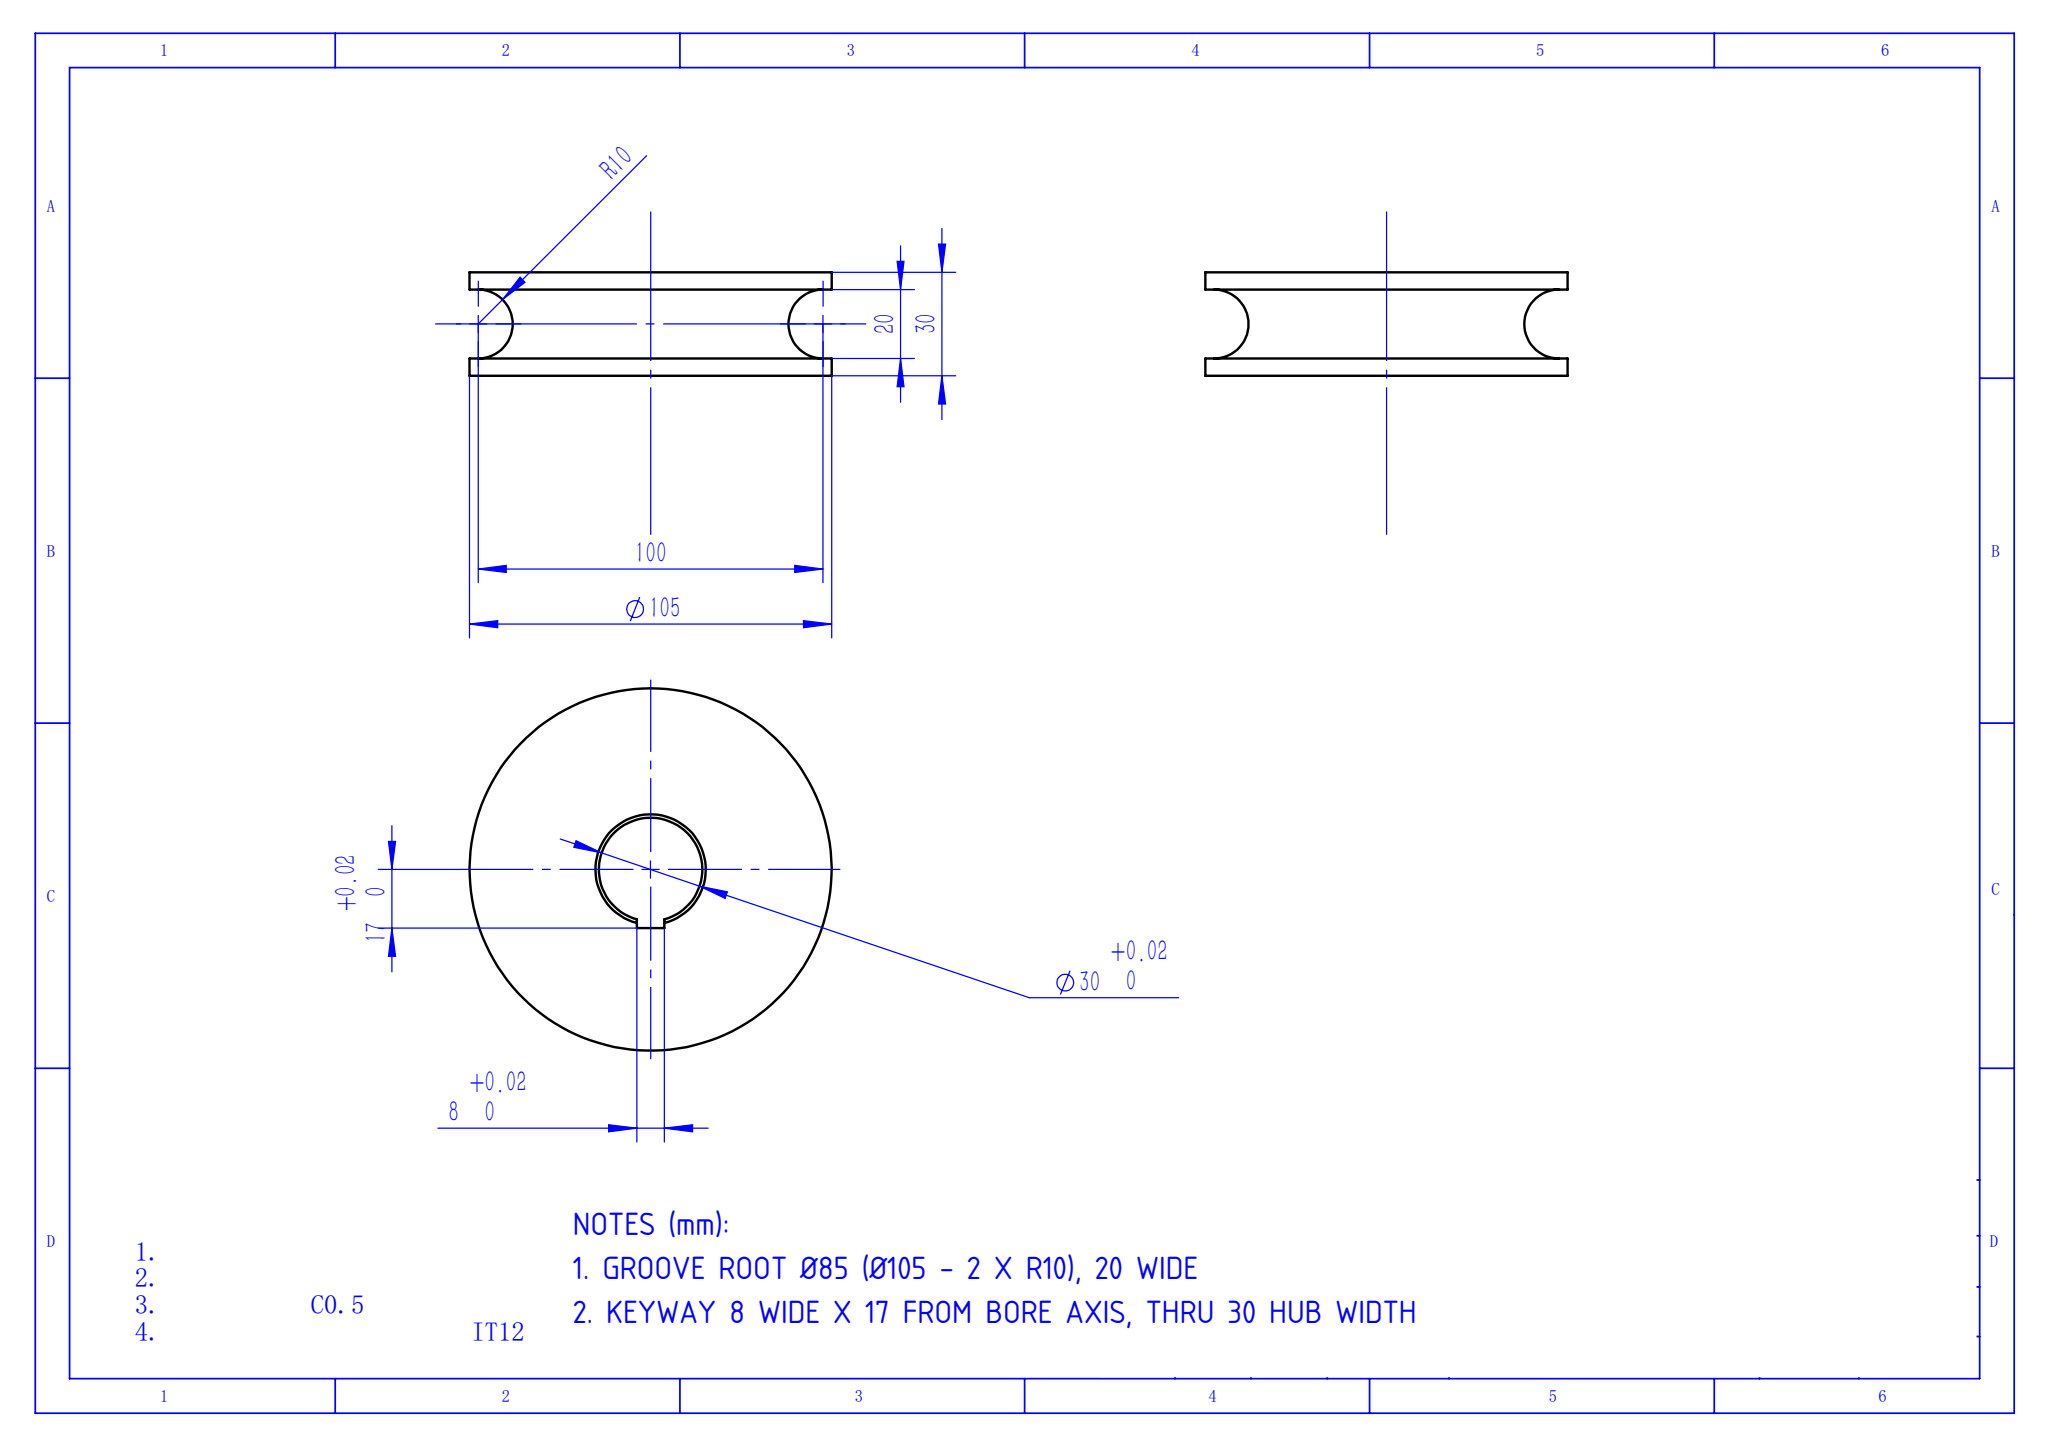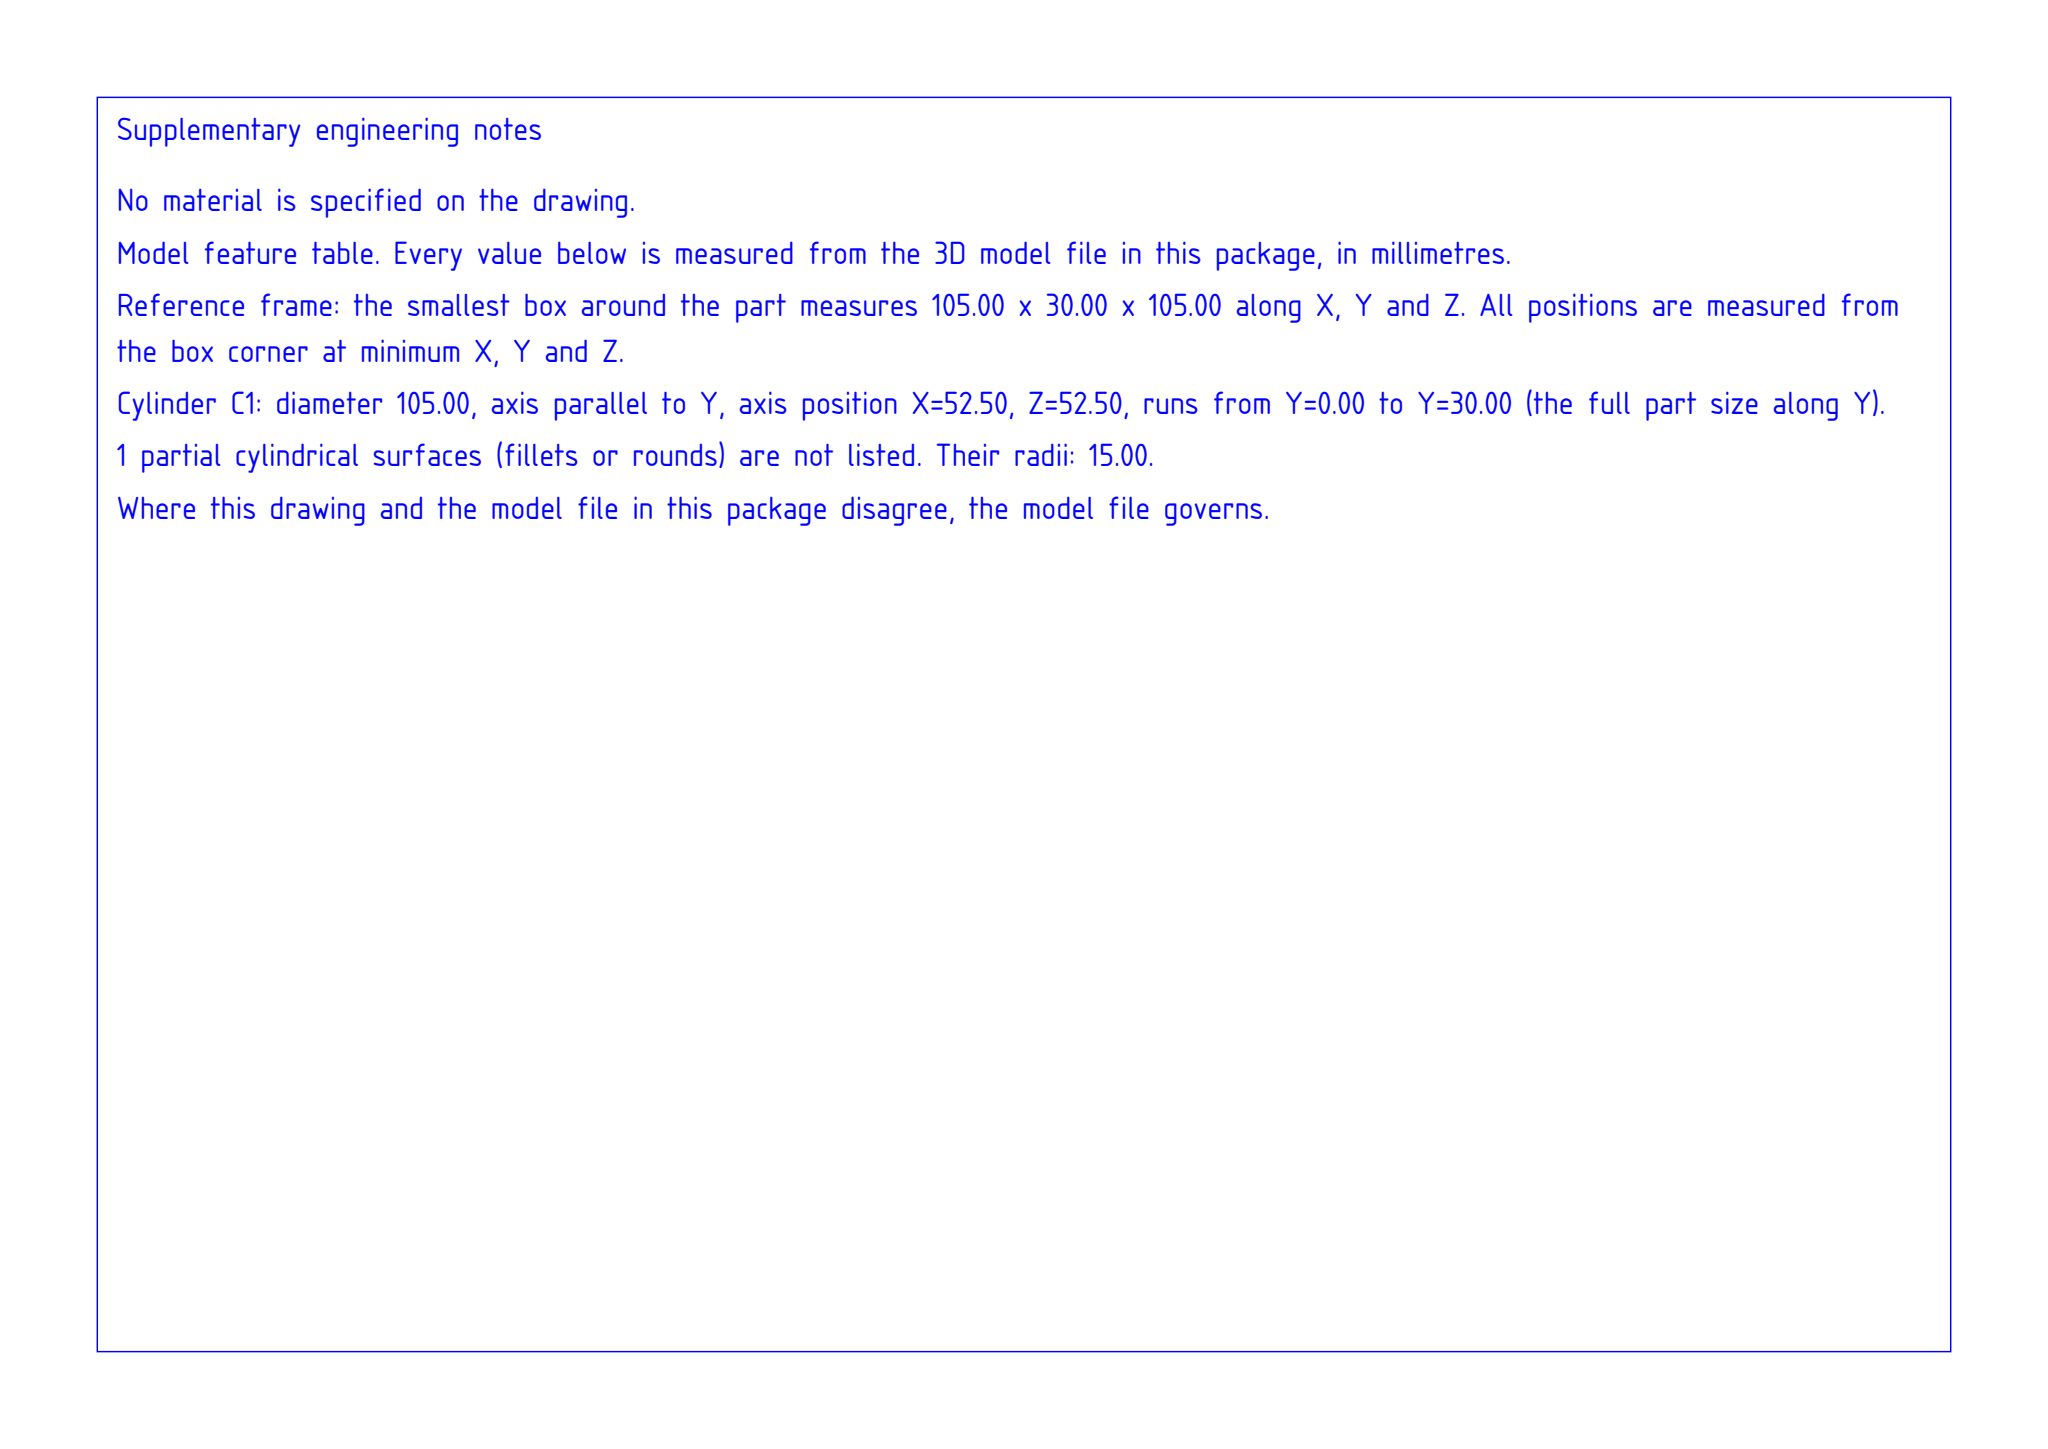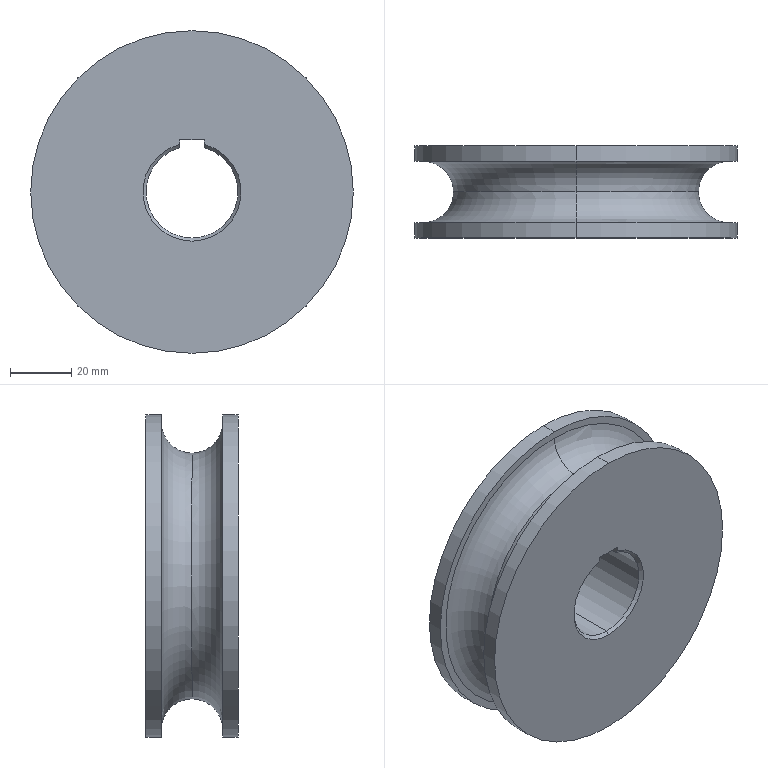Part | SolidWorks | mm | 1 solid | 20 faces | box 105 x 30 x 105 mm | volume 176693 mm3 | plane 7 | cylinder 6 | torus 4 | cone 3 | commonest cylinder face diameters 105 x4 30 x2
Drawing notes:
GROOVE ROOT Ø85 (Ø105 - 2 X R10), 20 WIDE | from the solid: Ø105 outer cyl with 4 x R10 fillets forming groove between y=5 and y=25 (20 wide); 105-2(10)=85
KEYWAY 8 WIDE X 17 FROM BORE AXIS, THRU 30 HUB WIDTH | from the solid: x-planes 57.8 & 65.8 (8 wide, ctr 61.8), z-plane 78.8 = 17 from axis z=61.8, spans y=0 to y=30
build123d program:
from build123d import *

# Parameters (mm, degrees)
CHAMFER1_SIZE = 1
KEYWAY_DEPTH  = 96.118


with BuildPart() as part:
    # Sketch1 → Revolve1 (revolve)
    with BuildSketch(Plane.XY, mode=Mode.PRIVATE) as revolve1_sk:
        with BuildLine():
            Line((15, -15), (52.5, -15))
            Line((52.5, -15), (52.5, -10))
            Line((52.5, -10), (50, -10))
            ThreePointArc((50, -10), (40, 0), (50, 10))
            Line((50, 10), (52.5, 10))
            Line((52.5, 10), (52.5, 15))
            Line((52.5, 15), (15, 15))
            Line((15, 15), (15, -15))
        make_face()
    revolve(revolve1_sk.sketch.rotate(Axis((0, 0, 0), (0, 1, 0)), 90), axis=Axis((0, 0, 0), (0, 1, 0)))

    # Chamfer1
    chamfer1_edges = [part.edges().sort_by_distance(p)[0] for p in [
        (0, -15, 15),
        (0, 15, 15),
    ]]
    chamfer(chamfer1_edges, length=CHAMFER1_SIZE)

    # KeySketch → Keyway (cut, through all)
    with BuildSketch(Plane(origin=(-16.943, 15, 5.163), x_dir=(-1, 0, 0), z_dir=(0, 1, 0))):
        with BuildLine():
            Line((-20.943, 9.294), (-20.943, 11.837))
            Line((-20.943, 11.837), (-12.943, 11.837))
            Line((-12.943, 11.837), (-12.943, 9.294))
            ThreePointArc((-12.943, 9.294), (-16.943, -20.163), (-20.943, 9.294))
        make_face()
    extrude(amount=-KEYWAY_DEPTH, mode=Mode.SUBTRACT)


solid = part.part
STEP:
#1=CARTESIAN_POINT('',(0.,-10.,-50.));
#2=VERTEX_POINT('',#1);
#3=CARTESIAN_POINT('',(0.,0.,-40.));
#4=VERTEX_POINT('',#3);
#5=CARTESIAN_POINT('',(0.,0.,-50.));
#6=DIRECTION('',(-1.,0.,0.));
#7=DIRECTION('',(0.,0.,1.));
#8=AXIS2_PLACEMENT_3D('',#5,#6,#7);
#9=CIRCLE('',#8,10.);
#10=EDGE_CURVE('',#2,#4,#9,.T.);
#11=ORIENTED_EDGE('',*,*,#10,.T.);
#12=CARTESIAN_POINT('',(0.,0.,40.));
#13=VERTEX_POINT('',#12);
#14=CARTESIAN_POINT('',(0.,0.,0.));
#15=DIRECTION('',(0.,-1.,0.));
#16=DIRECTION('',(0.,0.,-1.));
#17=AXIS2_PLACEMENT_3D('',#14,#15,#16);
#18=CIRCLE('',#17,40.);
#19=EDGE_CURVE('',#4,#13,#18,.T.);
#20=ORIENTED_EDGE('',*,*,#19,.T.);
#21=CARTESIAN_POINT('',(0.,-10.,50.));
#22=VERTEX_POINT('',#21);
#23=CARTESIAN_POINT('',(0.,0.,50.));
#24=DIRECTION('',(1.,0.,-0.));
#25=DIRECTION('',(-0.,0.,-1.));
#26=AXIS2_PLACEMENT_3D('',#23,#24,#25);
#27=CIRCLE('',#26,10.);
#28=EDGE_CURVE('',#22,#13,#27,.T.);
#29=ORIENTED_EDGE('',*,*,#28,.F.);
#30=CARTESIAN_POINT('',(0.,-10.,0.));
#31=DIRECTION('',(0.,-1.,0.));
#32=DIRECTION('',(0.,0.,-1.));
#33=AXIS2_PLACEMENT_3D('',#30,#31,#32);
#34=CIRCLE('',#33,50.);
#35=EDGE_CURVE('',#2,#22,#34,.T.);
#36=ORIENTED_EDGE('',*,*,#35,.F.);
#37=EDGE_LOOP('',(#11,#20,#29,#36));
#38=FACE_OUTER_BOUND('',#37,.T.);
#39=CARTESIAN_POINT('',(0.,0.,0.));
#40=DIRECTION('',(0.,-1.,0.));
#41=DIRECTION('',(0.,0.,-1.));
#42=AXIS2_PLACEMENT_3D('',#39,#40,#41);
#43=TOROIDAL_SURFACE('',#42,50.,10.);
#44=ADVANCED_FACE('',(#38),#43,.F.);
#45=ORIENTED_EDGE('',*,*,#28,.T.);
#46=CARTESIAN_POINT('',(0.,0.,0.));
#47=DIRECTION('',(0.,-1.,0.));
#48=DIRECTION('',(0.,0.,-1.));
#49=AXIS2_PLACEMENT_3D('',#46,#47,#48);
#50=CIRCLE('',#49,40.);
#51=EDGE_CURVE('',#13,#4,#50,.T.);
#52=ORIENTED_EDGE('',*,*,#51,.T.);
#53=ORIENTED_EDGE('',*,*,#10,.F.);
#54=CARTESIAN_POINT('',(0.,-10.,0.));
#55=DIRECTION('',(0.,-1.,0.));
#56=DIRECTION('',(0.,0.,-1.));
#57=AXIS2_PLACEMENT_3D('',#54,#55,#56);
#58=CIRCLE('',#57,50.);
#59=EDGE_CURVE('',#22,#2,#58,.T.);
#60=ORIENTED_EDGE('',*,*,#59,.F.);
#61=EDGE_LOOP('',(#45,#52,#53,#60));
#62=FACE_OUTER_BOUND('',#61,.T.);
#63=CARTESIAN_POINT('',(0.,0.,0.));
#64=DIRECTION('',(0.,-1.,0.));
#65=DIRECTION('',(0.,0.,-1.));
#66=AXIS2_PLACEMENT_3D('',#63,#64,#65);
#67=TOROIDAL_SURFACE('',#66,50.,10.);
#68=ADVANCED_FACE('',(#62),#67,.F.);
#69=CARTESIAN_POINT('',(0.,15.,-52.5));
#70=VERTEX_POINT('',#69);
#71=CARTESIAN_POINT('',(0.,15.,52.5));
#72=VERTEX_POINT('',#71);
#73=CARTESIAN_POINT('',(0.,15.,0.));
#74=DIRECTION('',(0.,-1.,0.));
#75=DIRECTION('',(0.,0.,-1.));
#76=AXIS2_PLACEMENT_3D('',#73,#74,#75);
#77=CIRCLE('',#76,52.5);
#78=EDGE_CURVE('',#70,#72,#77,.T.);
#79=ORIENTED_EDGE('',*,*,#78,.T.);
#80=CARTESIAN_POINT('',(0.,10.,52.5));
#81=VERTEX_POINT('',#80);
#82=CARTESIAN_POINT('',(0.,0.,52.5));
#83=DIRECTION('',(0.,-1.,0.));
#84=VECTOR('',#83,1000.);
#85=LINE('',#82,#84);
#86=EDGE_CURVE('',#72,#81,#85,.T.);
#87=ORIENTED_EDGE('',*,*,#86,.T.);
#88=CARTESIAN_POINT('',(0.,10.,-52.5));
#89=VERTEX_POINT('',#88);
#90=CARTESIAN_POINT('',(0.,10.,0.));
#91=DIRECTION('',(0.,-1.,0.));
#92=DIRECTION('',(0.,0.,-1.));
#93=AXIS2_PLACEMENT_3D('',#90,#91,#92);
#94=CIRCLE('',#93,52.5);
#95=EDGE_CURVE('',#89,#81,#94,.T.);
#96=ORIENTED_EDGE('',*,*,#95,.F.);
#97=CARTESIAN_POINT('',(0.,0.,-52.5));
#98=DIRECTION('',(0.,-1.,0.));
#99=VECTOR('',#98,1000.);
#100=LINE('',#97,#99);
#101=EDGE_CURVE('',#70,#89,#100,.T.);
#102=ORIENTED_EDGE('',*,*,#101,.F.);
#103=EDGE_LOOP('',(#79,#87,#96,#102));
#104=FACE_OUTER_BOUND('',#103,.T.);
#105=CARTESIAN_POINT('',(0.,0.,0.));
#106=DIRECTION('',(0.,-1.,0.));
#107=DIRECTION('',(0.,0.,-1.));
#108=AXIS2_PLACEMENT_3D('',#105,#106,#107);
#109=CYLINDRICAL_SURFACE('',#108,52.5);
#110=ADVANCED_FACE('',(#104),#109,.T.);
#111=ORIENTED_EDGE('',*,*,#51,.F.);
#112=CARTESIAN_POINT('',(0.,10.,50.));
#113=VERTEX_POINT('',#112);
#114=CARTESIAN_POINT('',(0.,0.,50.));
#115=DIRECTION('',(1.,0.,-0.));
#116=DIRECTION('',(-0.,0.,-1.));
#117=AXIS2_PLACEMENT_3D('',#114,#115,#116);
#118=CIRCLE('',#117,10.);
#119=EDGE_CURVE('',#13,#113,#118,.T.);
#120=ORIENTED_EDGE('',*,*,#119,.T.);
#121=CARTESIAN_POINT('',(0.,10.,-50.));
#122=VERTEX_POINT('',#121);
#123=CARTESIAN_POINT('',(0.,10.,0.));
#124=DIRECTION('',(0.,-1.,0.));
#125=DIRECTION('',(0.,0.,-1.));
#126=AXIS2_PLACEMENT_3D('',#123,#124,#125);
#127=CIRCLE('',#126,50.);
#128=EDGE_CURVE('',#113,#122,#127,.T.);
#129=ORIENTED_EDGE('',*,*,#128,.T.);
#130=CARTESIAN_POINT('',(0.,0.,-50.));
#131=DIRECTION('',(-1.,0.,0.));
#132=DIRECTION('',(0.,0.,1.));
#133=AXIS2_PLACEMENT_3D('',#130,#131,#132);
#134=CIRCLE('',#133,10.);
#135=EDGE_CURVE('',#4,#122,#134,.T.);
#136=ORIENTED_EDGE('',*,*,#135,.F.);
#137=EDGE_LOOP('',(#111,#120,#129,#136));
#138=FACE_OUTER_BOUND('',#137,.T.);
#139=CARTESIAN_POINT('',(0.,0.,0.));
#140=DIRECTION('',(0.,-1.,0.));
#141=DIRECTION('',(0.,0.,-1.));
#142=AXIS2_PLACEMENT_3D('',#139,#140,#141);
#143=TOROIDAL_SURFACE('',#142,50.,10.);
#144=ADVANCED_FACE('',(#138),#143,.F.);
#145=CARTESIAN_POINT('',(0.,-10.,-52.5));
#146=VERTEX_POINT('',#145);
#147=CARTESIAN_POINT('',(0.,-10.,52.5));
#148=VERTEX_POINT('',#147);
#149=CARTESIAN_POINT('',(0.,-10.,0.));
#150=DIRECTION('',(0.,-1.,0.));
#151=DIRECTION('',(0.,0.,-1.));
#152=AXIS2_PLACEMENT_3D('',#149,#150,#151);
#153=CIRCLE('',#152,52.5);
#154=EDGE_CURVE('',#146,#148,#153,.T.);
#155=ORIENTED_EDGE('',*,*,#154,.T.);
#156=CARTESIAN_POINT('',(0.,-15.,52.5));
#157=VERTEX_POINT('',#156);
#158=CARTESIAN_POINT('',(0.,0.,52.5));
#159=DIRECTION('',(0.,-1.,0.));
#160=VECTOR('',#159,1000.);
#161=LINE('',#158,#160);
#162=EDGE_CURVE('',#148,#157,#161,.T.);
#163=ORIENTED_EDGE('',*,*,#162,.T.);
#164=CARTESIAN_POINT('',(0.,-15.,-52.5));
#165=VERTEX_POINT('',#164);
#166=CARTESIAN_POINT('',(0.,-15.,0.));
#167=DIRECTION('',(0.,-1.,0.));
#168=DIRECTION('',(0.,0.,-1.));
#169=AXIS2_PLACEMENT_3D('',#166,#167,#168);
#170=CIRCLE('',#169,52.5);
#171=EDGE_CURVE('',#165,#157,#170,.T.);
#172=ORIENTED_EDGE('',*,*,#171,.F.);
#173=CARTESIAN_POINT('',(0.,0.,-52.5));
#174=DIRECTION('',(0.,-1.,0.));
#175=VECTOR('',#174,1000.);
#176=LINE('',#173,#175);
#177=EDGE_CURVE('',#146,#165,#176,.T.);
#178=ORIENTED_EDGE('',*,*,#177,.F.);
#179=EDGE_LOOP('',(#155,#163,#172,#178));
#180=FACE_OUTER_BOUND('',#179,.T.);
#181=CARTESIAN_POINT('',(0.,0.,0.));
#182=DIRECTION('',(0.,-1.,0.));
#183=DIRECTION('',(0.,0.,-1.));
#184=AXIS2_PLACEMENT_3D('',#181,#182,#183);
#185=CYLINDRICAL_SURFACE('',#184,52.5);
#186=ADVANCED_FACE('',(#180),#185,.T.);
#187=CARTESIAN_POINT('',(0.,-14.,-15.));
#188=VERTEX_POINT('',#187);
#189=CARTESIAN_POINT('',(4.,-14.,14.457));
#190=VERTEX_POINT('',#189);
#191=CARTESIAN_POINT('',(0.,-14.,0.));
#192=DIRECTION('',(0.,-1.,0.));
#193=DIRECTION('',(0.,0.,-1.));
#194=AXIS2_PLACEMENT_3D('',#191,#192,#193);
#195=CIRCLE('',#194,15.);
#196=EDGE_CURVE('',#188,#190,#195,.T.);
#197=ORIENTED_EDGE('',*,*,#196,.F.);
#198=CARTESIAN_POINT('',(0.,-15.,-16.));
#199=VERTEX_POINT('',#198);
#200=CARTESIAN_POINT('',(0.,-14.,-15.));
#201=DIRECTION('',(0.,-0.7071,-0.7071));
#202=VECTOR('',#201,1000.);
#203=LINE('',#200,#202);
#204=EDGE_CURVE('',#188,#199,#203,.T.);
#205=ORIENTED_EDGE('',*,*,#204,.T.);
#206=CARTESIAN_POINT('',(4.,-15.,15.492));
#207=VERTEX_POINT('',#206);
#208=CARTESIAN_POINT('',(0.,-15.,0.));
#209=DIRECTION('',(0.,1.,0.));
#210=DIRECTION('',(0.,0.,-1.));
#211=AXIS2_PLACEMENT_3D('',#208,#209,#210);
#212=CIRCLE('',#211,16.);
#213=EDGE_CURVE('',#207,#199,#212,.T.);
#214=ORIENTED_EDGE('',*,*,#213,.F.);
#215=CARTESIAN_POINT('',(4.,-15.,15.492));
#216=CARTESIAN_POINT('',(4.,-14.666,15.147));
#217=CARTESIAN_POINT('',(4.,-14.333,14.802));
#218=CARTESIAN_POINT('',(4.,-14.,14.457));
#219=B_SPLINE_CURVE_WITH_KNOTS('',3,(#215,#216,#217,#218),.UNSPECIFIED.,.F.,.F.,(4,4),(0.003063,0.004502),.UNSPECIFIED.);
#220=EDGE_CURVE('',#207,#190,#219,.T.);
#221=ORIENTED_EDGE('',*,*,#220,.T.);
#222=EDGE_LOOP('',(#197,#205,#214,#221));
#223=FACE_OUTER_BOUND('',#222,.T.);
#224=CARTESIAN_POINT('',(0.,-14.,0.));
#225=DIRECTION('',(0.,-1.,0.));
#226=DIRECTION('',(0.,0.,-1.));
#227=AXIS2_PLACEMENT_3D('',#224,#225,#226);
#228=CONICAL_SURFACE('',#227,15.,0.7854);
#229=ADVANCED_FACE('',(#223),#228,.F.);
#230=CARTESIAN_POINT('',(4.,14.,14.457));
#231=VERTEX_POINT('',#230);
#232=CARTESIAN_POINT('',(0.,14.,-15.));
#233=VERTEX_POINT('',#232);
#234=CARTESIAN_POINT('',(0.,14.,0.));
#235=DIRECTION('',(0.,1.,0.));
#236=DIRECTION('',(0.,0.,1.));
#237=AXIS2_PLACEMENT_3D('',#234,#235,#236);
#238=CIRCLE('',#237,15.);
#239=EDGE_CURVE('',#231,#233,#238,.T.);
#240=ORIENTED_EDGE('',*,*,#239,.T.);
#241=CARTESIAN_POINT('',(0.,0.,-15.));
#242=DIRECTION('',(0.,-1.,0.));
#243=VECTOR('',#242,1000.);
#244=LINE('',#241,#243);
#245=EDGE_CURVE('',#233,#188,#244,.T.);
#246=ORIENTED_EDGE('',*,*,#245,.T.);
#247=ORIENTED_EDGE('',*,*,#196,.T.);
#248=CARTESIAN_POINT('',(4.,-15.,14.457));
#249=DIRECTION('',(0.,1.,0.));
#250=VECTOR('',#249,1000.);
#251=LINE('',#248,#250);
#252=EDGE_CURVE('',#190,#231,#251,.T.);
#253=ORIENTED_EDGE('',*,*,#252,.T.);
#254=EDGE_LOOP('',(#240,#246,#247,#253));
#255=FACE_OUTER_BOUND('',#254,.T.);
#256=CARTESIAN_POINT('',(0.,0.,0.));
#257=DIRECTION('',(0.,-1.,0.));
#258=DIRECTION('',(0.,0.,-1.));
#259=AXIS2_PLACEMENT_3D('',#256,#257,#258);
#260=CYLINDRICAL_SURFACE('',#259,15.);
#261=ADVANCED_FACE('',(#255),#260,.F.);
#262=ORIENTED_EDGE('',*,*,#245,.F.);
#263=CARTESIAN_POINT('',(-4.,14.,14.457));
#264=VERTEX_POINT('',#263);
#265=CARTESIAN_POINT('',(0.,14.,0.));
#266=DIRECTION('',(0.,1.,0.));
#267=DIRECTION('',(0.,0.,1.));
#268=AXIS2_PLACEMENT_3D('',#265,#266,#267);
#269=CIRCLE('',#268,15.);
#270=EDGE_CURVE('',#233,#264,#269,.T.);
#271=ORIENTED_EDGE('',*,*,#270,.T.);
#272=CARTESIAN_POINT('',(-4.,-14.,14.457));
#273=VERTEX_POINT('',#272);
#274=CARTESIAN_POINT('',(-4.,-15.,14.457));
#275=DIRECTION('',(0.,1.,0.));
#276=VECTOR('',#275,1000.);
#277=LINE('',#274,#276);
#278=EDGE_CURVE('',#273,#264,#277,.T.);
#279=ORIENTED_EDGE('',*,*,#278,.F.);
#280=CARTESIAN_POINT('',(0.,-14.,0.));
#281=DIRECTION('',(0.,-1.,0.));
#282=DIRECTION('',(0.,0.,-1.));
#283=AXIS2_PLACEMENT_3D('',#280,#281,#282);
#284=CIRCLE('',#283,15.);
#285=EDGE_CURVE('',#273,#188,#284,.T.);
#286=ORIENTED_EDGE('',*,*,#285,.T.);
#287=EDGE_LOOP('',(#262,#271,#279,#286));
#288=FACE_OUTER_BOUND('',#287,.T.);
#289=CARTESIAN_POINT('',(0.,0.,0.));
#290=DIRECTION('',(0.,-1.,0.));
#291=DIRECTION('',(0.,0.,-1.));
#292=AXIS2_PLACEMENT_3D('',#289,#290,#291);
#293=CYLINDRICAL_SURFACE('',#292,15.);
#294=ADVANCED_FACE('',(#288),#293,.F.);
#295=ORIENTED_EDGE('',*,*,#171,.T.);
#296=CARTESIAN_POINT('',(0.,-15.,0.));
#297=DIRECTION('',(0.,-1.,0.));
#298=DIRECTION('',(0.,0.,-1.));
#299=AXIS2_PLACEMENT_3D('',#296,#297,#298);
#300=CIRCLE('',#299,52.5);
#301=EDGE_CURVE('',#157,#165,#300,.T.);
#302=ORIENTED_EDGE('',*,*,#301,.T.);
#303=EDGE_LOOP('',(#295,#302));
#304=FACE_OUTER_BOUND('',#303,.T.);
#305=ORIENTED_EDGE('',*,*,#213,.T.);
#306=CARTESIAN_POINT('',(-4.,-15.,15.492));
#307=VERTEX_POINT('',#306);
#308=CARTESIAN_POINT('',(0.,-15.,0.));
#309=DIRECTION('',(0.,1.,0.));
#310=DIRECTION('',(0.,0.,-1.));
#311=AXIS2_PLACEMENT_3D('',#308,#309,#310);
#312=CIRCLE('',#311,16.);
#313=EDGE_CURVE('',#199,#307,#312,.T.);
#314=ORIENTED_EDGE('',*,*,#313,.T.);
#315=CARTESIAN_POINT('',(-4.,-15.,17.));
#316=VERTEX_POINT('',#315);
#317=CARTESIAN_POINT('',(-4.,-15.,17.));
#318=DIRECTION('',(0.,0.,-1.));
#319=VECTOR('',#318,1000.);
#320=LINE('',#317,#319);
#321=EDGE_CURVE('',#316,#307,#320,.T.);
#322=ORIENTED_EDGE('',*,*,#321,.F.);
#323=CARTESIAN_POINT('',(4.,-15.,17.));
#324=VERTEX_POINT('',#323);
#325=CARTESIAN_POINT('',(-4.,-15.,17.));
#326=DIRECTION('',(1.,0.,0.));
#327=VECTOR('',#326,1000.);
#328=LINE('',#325,#327);
#329=EDGE_CURVE('',#316,#324,#328,.T.);
#330=ORIENTED_EDGE('',*,*,#329,.T.);
#331=CARTESIAN_POINT('',(4.,-15.,14.457));
#332=DIRECTION('',(0.,0.,1.));
#333=VECTOR('',#332,1000.);
#334=LINE('',#331,#333);
#335=EDGE_CURVE('',#207,#324,#334,.T.);
#336=ORIENTED_EDGE('',*,*,#335,.F.);
#337=EDGE_LOOP('',(#305,#314,#322,#330,#336));
#338=FACE_BOUND('',#337,.T.);
#339=CARTESIAN_POINT('',(15.,-15.,0.));
#340=DIRECTION('',(0.,-1.,0.));
#341=DIRECTION('',(0.,0.,-1.));
#342=AXIS2_PLACEMENT_3D('',#339,#340,#341);
#343=PLANE('',#342);
#344=ADVANCED_FACE('',(#304,#338),#343,.T.);
#345=ORIENTED_EDGE('',*,*,#78,.F.);
#346=CARTESIAN_POINT('',(0.,15.,0.));
#347=DIRECTION('',(0.,-1.,0.));
#348=DIRECTION('',(0.,0.,-1.));
#349=AXIS2_PLACEMENT_3D('',#346,#347,#348);
#350=CIRCLE('',#349,52.5);
#351=EDGE_CURVE('',#72,#70,#350,.T.);
#352=ORIENTED_EDGE('',*,*,#351,.F.);
#353=EDGE_LOOP('',(#345,#352));
#354=FACE_OUTER_BOUND('',#353,.T.);
#355=CARTESIAN_POINT('',(-4.,15.,17.));
#356=VERTEX_POINT('',#355);
#357=CARTESIAN_POINT('',(4.,15.,17.));
#358=VERTEX_POINT('',#357);
#359=CARTESIAN_POINT('',(-4.,15.,17.));
#360=DIRECTION('',(1.,0.,0.));
#361=VECTOR('',#360,1000.);
#362=LINE('',#359,#361);
#363=EDGE_CURVE('',#356,#358,#362,.T.);
#364=ORIENTED_EDGE('',*,*,#363,.F.);
#365=CARTESIAN_POINT('',(-4.,15.,15.492));
#366=VERTEX_POINT('',#365);
#367=CARTESIAN_POINT('',(-4.,15.,17.));
#368=DIRECTION('',(0.,0.,-1.));
#369=VECTOR('',#368,1000.);
#370=LINE('',#367,#369);
#371=EDGE_CURVE('',#356,#366,#370,.T.);
#372=ORIENTED_EDGE('',*,*,#371,.T.);
#373=CARTESIAN_POINT('',(4.,15.,15.492));
#374=VERTEX_POINT('',#373);
#375=CARTESIAN_POINT('',(0.,15.,0.));
#376=DIRECTION('',(0.,-1.,0.));
#377=DIRECTION('',(0.,0.,1.));
#378=AXIS2_PLACEMENT_3D('',#375,#376,#377);
#379=CIRCLE('',#378,16.);
#380=EDGE_CURVE('',#366,#374,#379,.T.);
#381=ORIENTED_EDGE('',*,*,#380,.T.);
#382=CARTESIAN_POINT('',(4.,15.,14.457));
#383=DIRECTION('',(0.,0.,1.));
#384=VECTOR('',#383,1000.);
#385=LINE('',#382,#384);
#386=EDGE_CURVE('',#374,#358,#385,.T.);
#387=ORIENTED_EDGE('',*,*,#386,.T.);
#388=EDGE_LOOP('',(#364,#372,#381,#387));
#389=FACE_BOUND('',#388,.T.);
#390=CARTESIAN_POINT('',(15.,15.,0.));
#391=DIRECTION('',(0.,1.,0.));
#392=DIRECTION('',(0.,0.,1.));
#393=AXIS2_PLACEMENT_3D('',#390,#391,#392);
#394=PLANE('',#393);
#395=ADVANCED_FACE('',(#354,#389),#394,.T.);
#396=ORIENTED_EDGE('',*,*,#380,.F.);
#397=CARTESIAN_POINT('',(-4.,15.,15.492));
#398=CARTESIAN_POINT('',(-4.,14.666,15.147));
#399=CARTESIAN_POINT('',(-4.,14.333,14.802));
#400=CARTESIAN_POINT('',(-4.,14.,14.457));
#401=B_SPLINE_CURVE_WITH_KNOTS('',3,(#397,#398,#399,#400),.UNSPECIFIED.,.F.,.F.,(4,4),(0.002438,0.003877),.UNSPECIFIED.);
#402=EDGE_CURVE('',#366,#264,#401,.T.);
#403=ORIENTED_EDGE('',*,*,#402,.T.);
#404=ORIENTED_EDGE('',*,*,#270,.F.);
#405=ORIENTED_EDGE('',*,*,#239,.F.);
#406=CARTESIAN_POINT('',(4.,14.,14.457));
#407=CARTESIAN_POINT('',(4.,14.333,14.802));
#408=CARTESIAN_POINT('',(4.,14.666,15.147));
#409=CARTESIAN_POINT('',(4.,15.,15.492));
#410=B_SPLINE_CURVE_WITH_KNOTS('',3,(#406,#407,#408,#409),.UNSPECIFIED.,.F.,.F.,(4,4),(0.003253,0.004692),.UNSPECIFIED.);
#411=EDGE_CURVE('',#231,#374,#410,.T.);
#412=ORIENTED_EDGE('',*,*,#411,.T.);
#413=EDGE_LOOP('',(#396,#403,#404,#405,#412));
#414=FACE_OUTER_BOUND('',#413,.T.);
#415=CARTESIAN_POINT('',(0.,15.,0.));
#416=DIRECTION('',(0.,1.,0.));
#417=DIRECTION('',(0.,0.,1.));
#418=AXIS2_PLACEMENT_3D('',#415,#416,#417);
#419=CONICAL_SURFACE('',#418,16.,0.7854);
#420=ADVANCED_FACE('',(#414),#419,.F.);
#421=ORIENTED_EDGE('',*,*,#204,.F.);
#422=ORIENTED_EDGE('',*,*,#285,.F.);
#423=CARTESIAN_POINT('',(-4.,-14.,14.457));
#424=CARTESIAN_POINT('',(-4.,-14.333,14.802));
#425=CARTESIAN_POINT('',(-4.,-14.666,15.147));
#426=CARTESIAN_POINT('',(-4.,-15.,15.492));
#427=B_SPLINE_CURVE_WITH_KNOTS('',3,(#423,#424,#425,#426),.UNSPECIFIED.,.F.,.F.,(4,4),(0.002628,0.004067),.UNSPECIFIED.);
#428=EDGE_CURVE('',#273,#307,#427,.T.);
#429=ORIENTED_EDGE('',*,*,#428,.T.);
#430=ORIENTED_EDGE('',*,*,#313,.F.);
#431=EDGE_LOOP('',(#421,#422,#429,#430));
#432=FACE_OUTER_BOUND('',#431,.T.);
#433=CARTESIAN_POINT('',(0.,-14.,0.));
#434=DIRECTION('',(0.,-1.,0.));
#435=DIRECTION('',(0.,0.,-1.));
#436=AXIS2_PLACEMENT_3D('',#433,#434,#435);
#437=CONICAL_SURFACE('',#436,15.,0.7854);
#438=ADVANCED_FACE('',(#432),#437,.F.);
#439=ORIENTED_EDGE('',*,*,#162,.F.);
#440=CARTESIAN_POINT('',(0.,-10.,0.));
#441=DIRECTION('',(0.,-1.,0.));
#442=DIRECTION('',(0.,0.,-1.));
#443=AXIS2_PLACEMENT_3D('',#440,#441,#442);
#444=CIRCLE('',#443,52.5);
#445=EDGE_CURVE('',#148,#146,#444,.T.);
#446=ORIENTED_EDGE('',*,*,#445,.T.);
#447=ORIENTED_EDGE('',*,*,#177,.T.);
#448=ORIENTED_EDGE('',*,*,#301,.F.);
#449=EDGE_LOOP('',(#439,#446,#447,#448));
#450=FACE_OUTER_BOUND('',#449,.T.);
#451=CARTESIAN_POINT('',(0.,0.,0.));
#452=DIRECTION('',(0.,-1.,0.));
#453=DIRECTION('',(0.,0.,-1.));
#454=AXIS2_PLACEMENT_3D('',#451,#452,#453);
#455=CYLINDRICAL_SURFACE('',#454,52.5);
#456=ADVANCED_FACE('',(#450),#455,.T.);
#457=ORIENTED_EDGE('',*,*,#35,.T.);
#458=ORIENTED_EDGE('',*,*,#59,.T.);
#459=EDGE_LOOP('',(#457,#458));
#460=FACE_BOUND('',#459,.T.);
#461=ORIENTED_EDGE('',*,*,#154,.F.);
#462=ORIENTED_EDGE('',*,*,#445,.F.);
#463=EDGE_LOOP('',(#461,#462));
#464=FACE_OUTER_BOUND('',#463,.T.);
#465=CARTESIAN_POINT('',(52.5,-10.,0.));
#466=DIRECTION('',(0.,1.,0.));
#467=DIRECTION('',(0.,0.,1.));
#468=AXIS2_PLACEMENT_3D('',#465,#466,#467);
#469=PLANE('',#468);
#470=ADVANCED_FACE('',(#460,#464),#469,.T.);
#471=ORIENTED_EDGE('',*,*,#19,.F.);
#472=ORIENTED_EDGE('',*,*,#135,.T.);
#473=CARTESIAN_POINT('',(0.,10.,0.));
#474=DIRECTION('',(0.,-1.,0.));
#475=DIRECTION('',(0.,0.,-1.));
#476=AXIS2_PLACEMENT_3D('',#473,#474,#475);
#477=CIRCLE('',#476,50.);
#478=EDGE_CURVE('',#122,#113,#477,.T.);
#479=ORIENTED_EDGE('',*,*,#478,.T.);
#480=ORIENTED_EDGE('',*,*,#119,.F.);
#481=EDGE_LOOP('',(#471,#472,#479,#480));
#482=FACE_OUTER_BOUND('',#481,.T.);
#483=CARTESIAN_POINT('',(0.,0.,0.));
#484=DIRECTION('',(0.,-1.,0.));
#485=DIRECTION('',(0.,0.,-1.));
#486=AXIS2_PLACEMENT_3D('',#483,#484,#485);
#487=TOROIDAL_SURFACE('',#486,50.,10.);
#488=ADVANCED_FACE('',(#482),#487,.F.);
#489=ORIENTED_EDGE('',*,*,#95,.T.);
#490=CARTESIAN_POINT('',(0.,10.,0.));
#491=DIRECTION('',(0.,-1.,0.));
#492=DIRECTION('',(0.,0.,-1.));
#493=AXIS2_PLACEMENT_3D('',#490,#491,#492);
#494=CIRCLE('',#493,52.5);
#495=EDGE_CURVE('',#81,#89,#494,.T.);
#496=ORIENTED_EDGE('',*,*,#495,.T.);
#497=EDGE_LOOP('',(#489,#496));
#498=FACE_OUTER_BOUND('',#497,.T.);
#499=ORIENTED_EDGE('',*,*,#478,.F.);
#500=ORIENTED_EDGE('',*,*,#128,.F.);
#501=EDGE_LOOP('',(#499,#500));
#502=FACE_BOUND('',#501,.T.);
#503=CARTESIAN_POINT('',(52.5,10.,0.));
#504=DIRECTION('',(0.,-1.,0.));
#505=DIRECTION('',(0.,0.,-1.));
#506=AXIS2_PLACEMENT_3D('',#503,#504,#505);
#507=PLANE('',#506);
#508=ADVANCED_FACE('',(#498,#502),#507,.T.);
#509=ORIENTED_EDGE('',*,*,#86,.F.);
#510=ORIENTED_EDGE('',*,*,#351,.T.);
#511=ORIENTED_EDGE('',*,*,#101,.T.);
#512=ORIENTED_EDGE('',*,*,#495,.F.);
#513=EDGE_LOOP('',(#509,#510,#511,#512));
#514=FACE_OUTER_BOUND('',#513,.T.);
#515=CARTESIAN_POINT('',(0.,0.,0.));
#516=DIRECTION('',(0.,-1.,0.));
#517=DIRECTION('',(0.,0.,-1.));
#518=AXIS2_PLACEMENT_3D('',#515,#516,#517);
#519=CYLINDRICAL_SURFACE('',#518,52.5);
#520=ADVANCED_FACE('',(#514),#519,.T.);
#521=ORIENTED_EDGE('',*,*,#363,.T.);
#522=CARTESIAN_POINT('',(4.,-15.,17.));
#523=DIRECTION('',(0.,1.,0.));
#524=VECTOR('',#523,1000.);
#525=LINE('',#522,#524);
#526=EDGE_CURVE('',#324,#358,#525,.T.);
#527=ORIENTED_EDGE('',*,*,#526,.F.);
#528=ORIENTED_EDGE('',*,*,#329,.F.);
#529=CARTESIAN_POINT('',(-4.,-15.,17.));
#530=DIRECTION('',(0.,1.,0.));
#531=VECTOR('',#530,1000.);
#532=LINE('',#529,#531);
#533=EDGE_CURVE('',#316,#356,#532,.T.);
#534=ORIENTED_EDGE('',*,*,#533,.T.);
#535=EDGE_LOOP('',(#521,#527,#528,#534));
#536=FACE_OUTER_BOUND('',#535,.T.);
#537=CARTESIAN_POINT('',(-4.,-15.,17.));
#538=DIRECTION('',(0.,0.,1.));
#539=DIRECTION('',(1.,0.,0.));
#540=AXIS2_PLACEMENT_3D('',#537,#538,#539);
#541=PLANE('',#540);
#542=ADVANCED_FACE('',(#536),#541,.F.);
#543=ORIENTED_EDGE('',*,*,#371,.F.);
#544=ORIENTED_EDGE('',*,*,#533,.F.);
#545=ORIENTED_EDGE('',*,*,#321,.T.);
#546=ORIENTED_EDGE('',*,*,#428,.F.);
#547=ORIENTED_EDGE('',*,*,#278,.T.);
#548=ORIENTED_EDGE('',*,*,#402,.F.);
#549=EDGE_LOOP('',(#543,#544,#545,#546,#547,#548));
#550=FACE_OUTER_BOUND('',#549,.T.);
#551=CARTESIAN_POINT('',(-4.,-15.,17.));
#552=DIRECTION('',(1.,0.,0.));
#553=DIRECTION('',(0.,0.,-1.));
#554=AXIS2_PLACEMENT_3D('',#551,#552,#553);
#555=PLANE('',#554);
#556=ADVANCED_FACE('',(#550),#555,.T.);
#557=ORIENTED_EDGE('',*,*,#252,.F.);
#558=ORIENTED_EDGE('',*,*,#220,.F.);
#559=ORIENTED_EDGE('',*,*,#335,.T.);
#560=ORIENTED_EDGE('',*,*,#526,.T.);
#561=ORIENTED_EDGE('',*,*,#386,.F.);
#562=ORIENTED_EDGE('',*,*,#411,.F.);
#563=EDGE_LOOP('',(#557,#558,#559,#560,#561,#562));
#564=FACE_OUTER_BOUND('',#563,.T.);
#565=CARTESIAN_POINT('',(4.,-15.,14.457));
#566=DIRECTION('',(-1.,0.,0.));
#567=DIRECTION('',(0.,0.,1.));
#568=AXIS2_PLACEMENT_3D('',#565,#566,#567);
#569=PLANE('',#568);
#570=ADVANCED_FACE('',(#564),#569,.T.);
#571=CLOSED_SHELL('',(#44,#68,#110,#144,#186,#229,#261,#294,#344,#395,#420,#438,#456,#470,#488,#508,#520,#542,#556,#570));
#572=MANIFOLD_SOLID_BREP('',#571);
#573=CARTESIAN_POINT('',(0.,0.,0.));
#574=DIRECTION('',(0.,0.,1.));
#575=DIRECTION('',(1.,0.,0.));
#576=AXIS2_PLACEMENT_3D('',#573,#574,#575);
#577=(LENGTH_UNIT()NAMED_UNIT(*)SI_UNIT(.MILLI.,.METRE.));
#578=UNCERTAINTY_MEASURE_WITH_UNIT(LENGTH_MEASURE(0.00001),#577,'','');
#579=(NAMED_UNIT(*)PLANE_ANGLE_UNIT()SI_UNIT($,.RADIAN.));
#580=(NAMED_UNIT(*)SI_UNIT($,.STERADIAN.)SOLID_ANGLE_UNIT());
#581=(GEOMETRIC_REPRESENTATION_CONTEXT(3)GLOBAL_UNCERTAINTY_ASSIGNED_CONTEXT((#578))GLOBAL_UNIT_ASSIGNED_CONTEXT((#577,#579,#580))REPRESENTATION_CONTEXT('',''));
#582=ADVANCED_BREP_SHAPE_REPRESENTATION('',(#572,#576),#581);